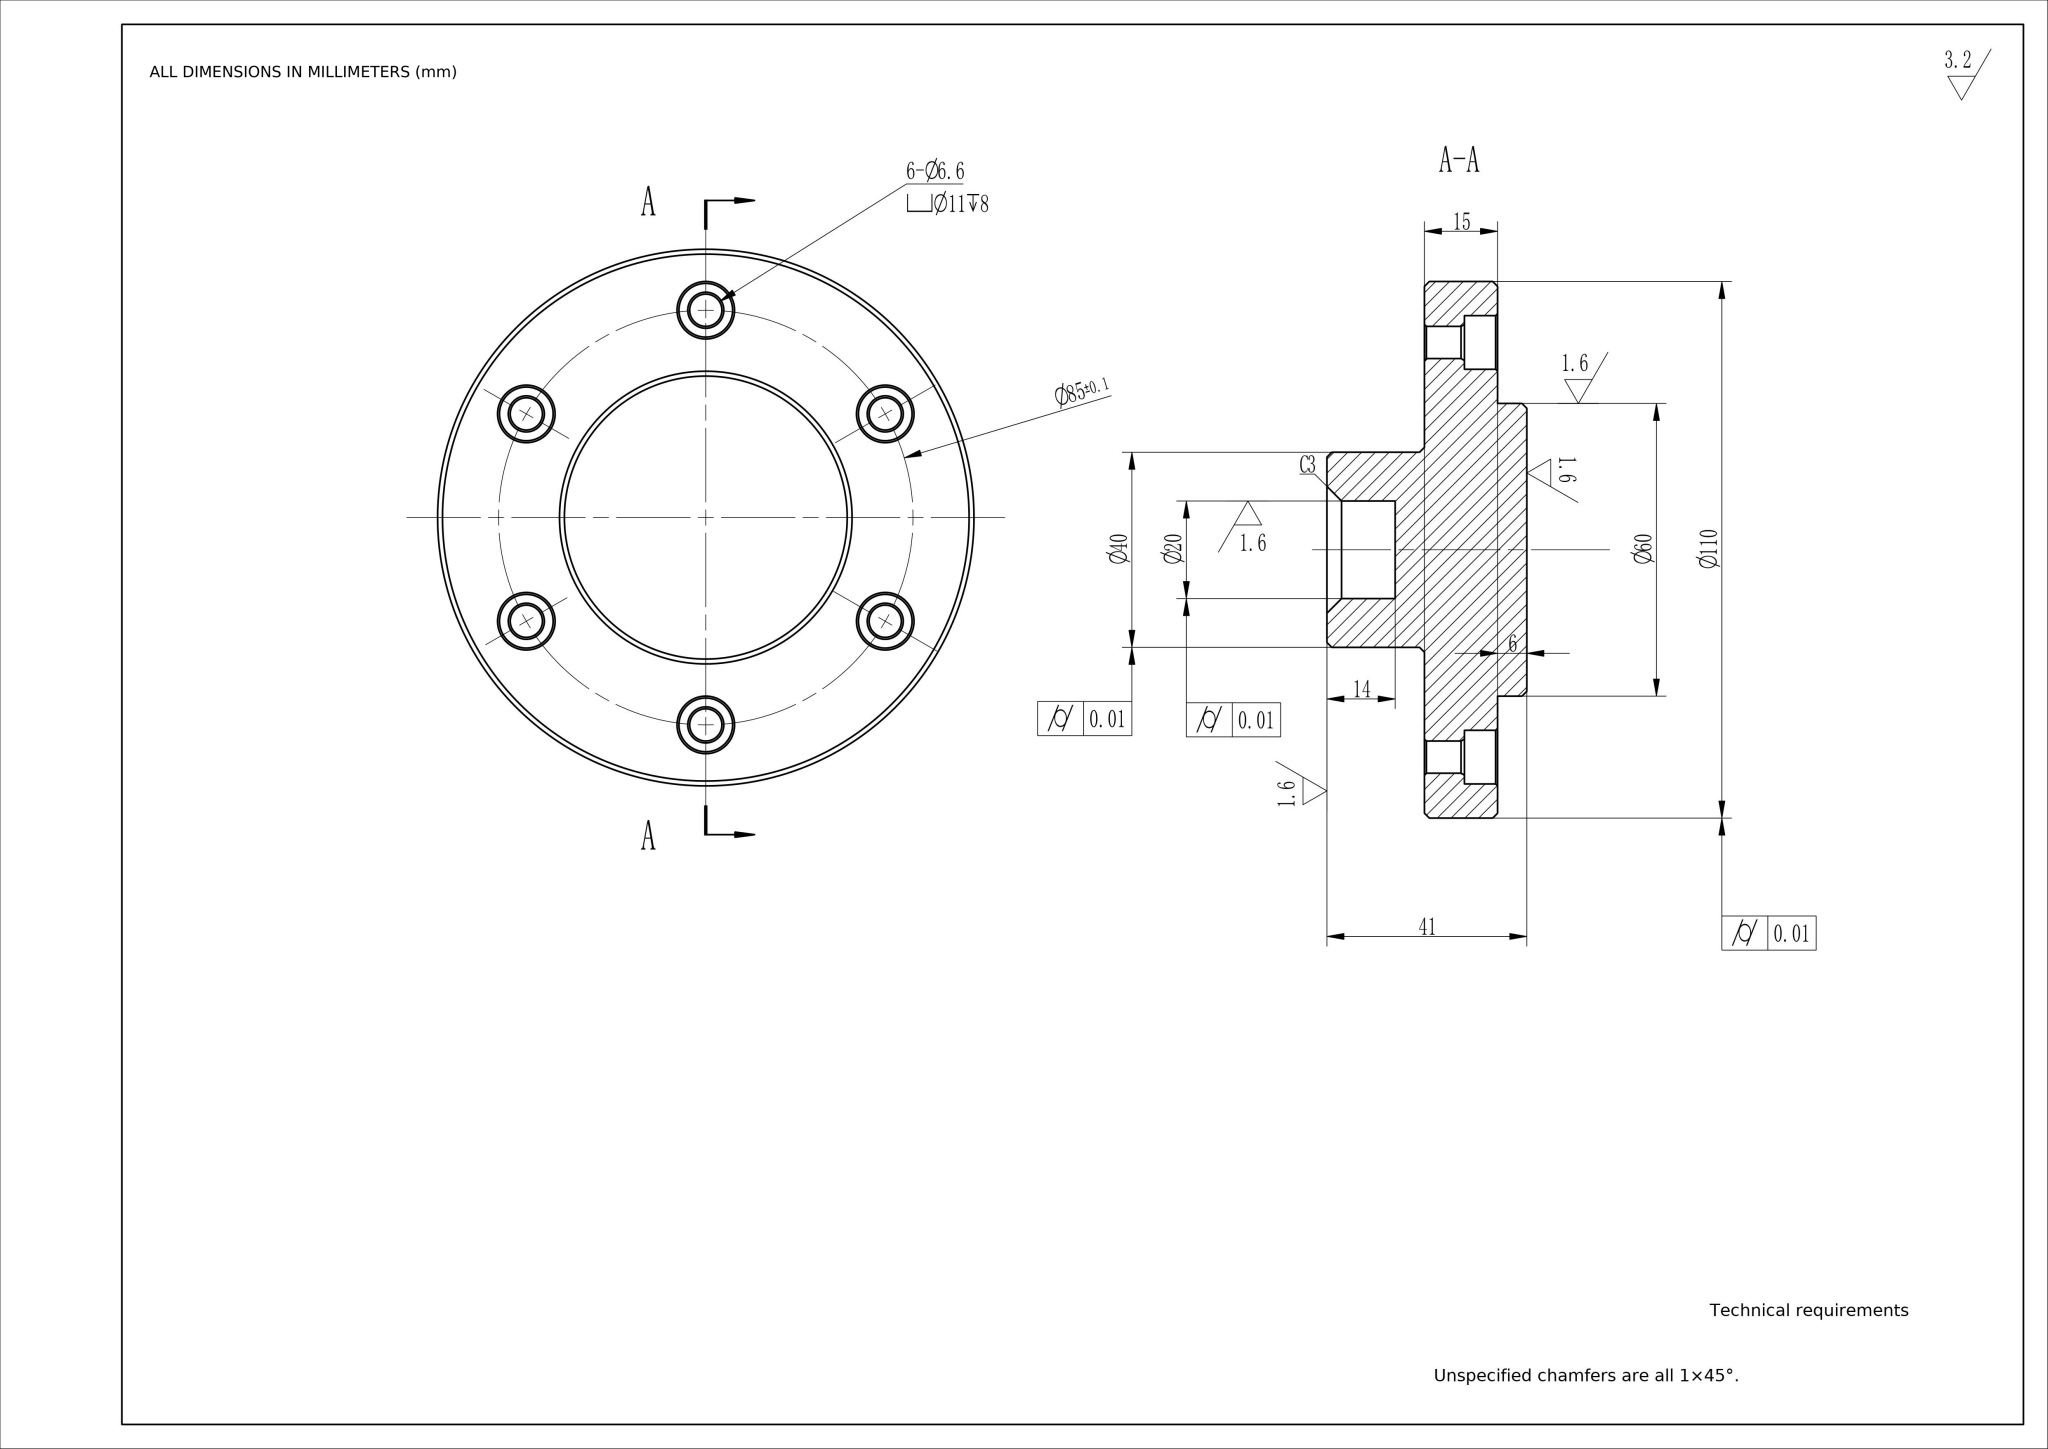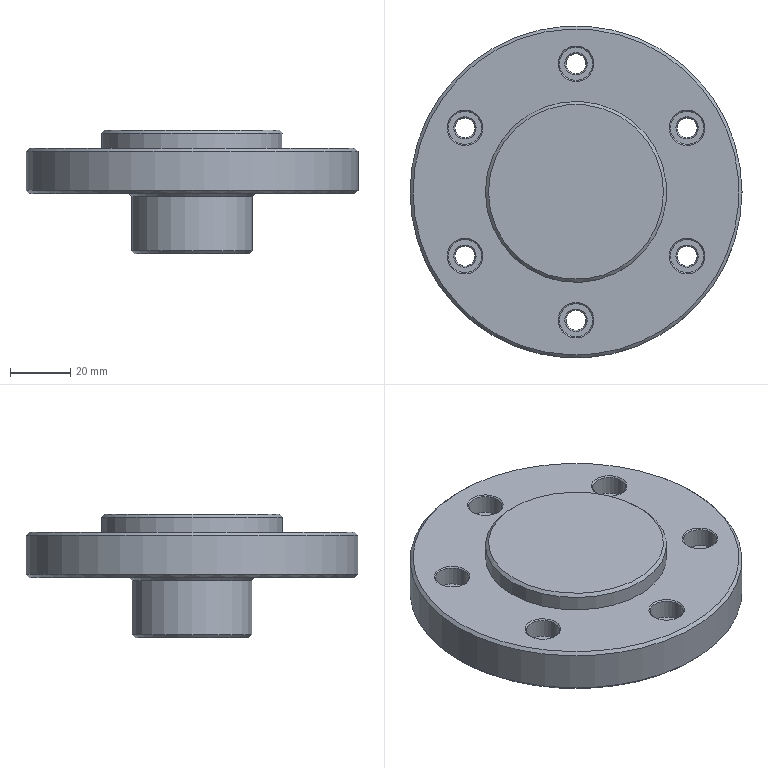Part | NX | mm | 1 solid | 51 faces | box 110 x 110 x 41 mm | volume 173897 mm3 | cone 24 | cylinder 16 | plane 11 | commonest cylinder face diameters 6.6 x6 11 x6 110 x1 40 x1 60 x1 20 x1